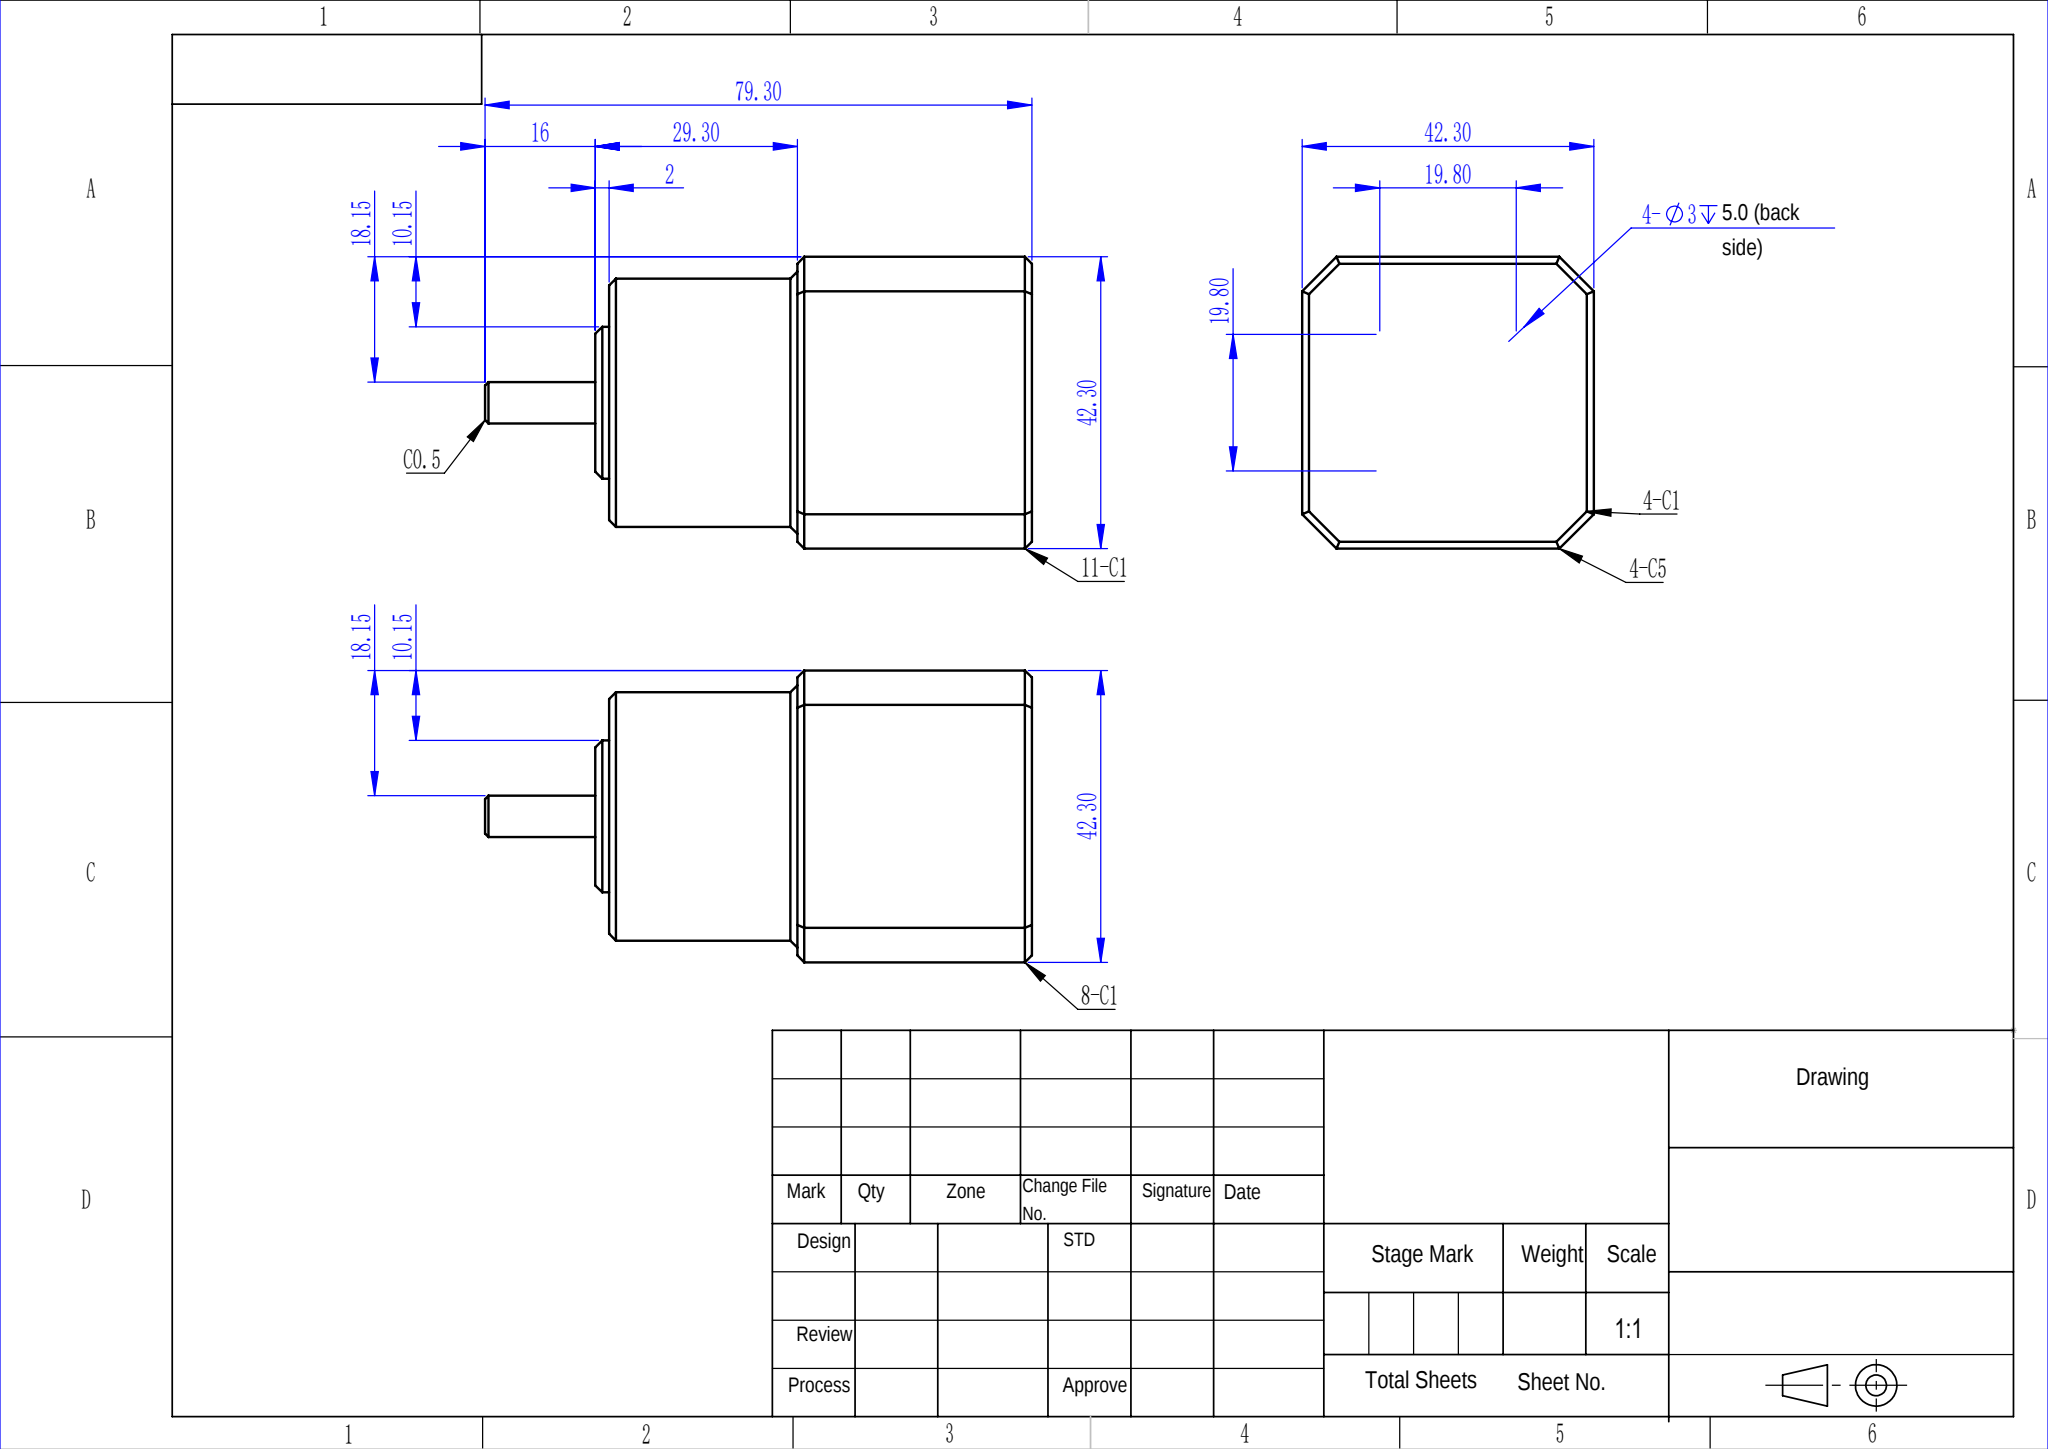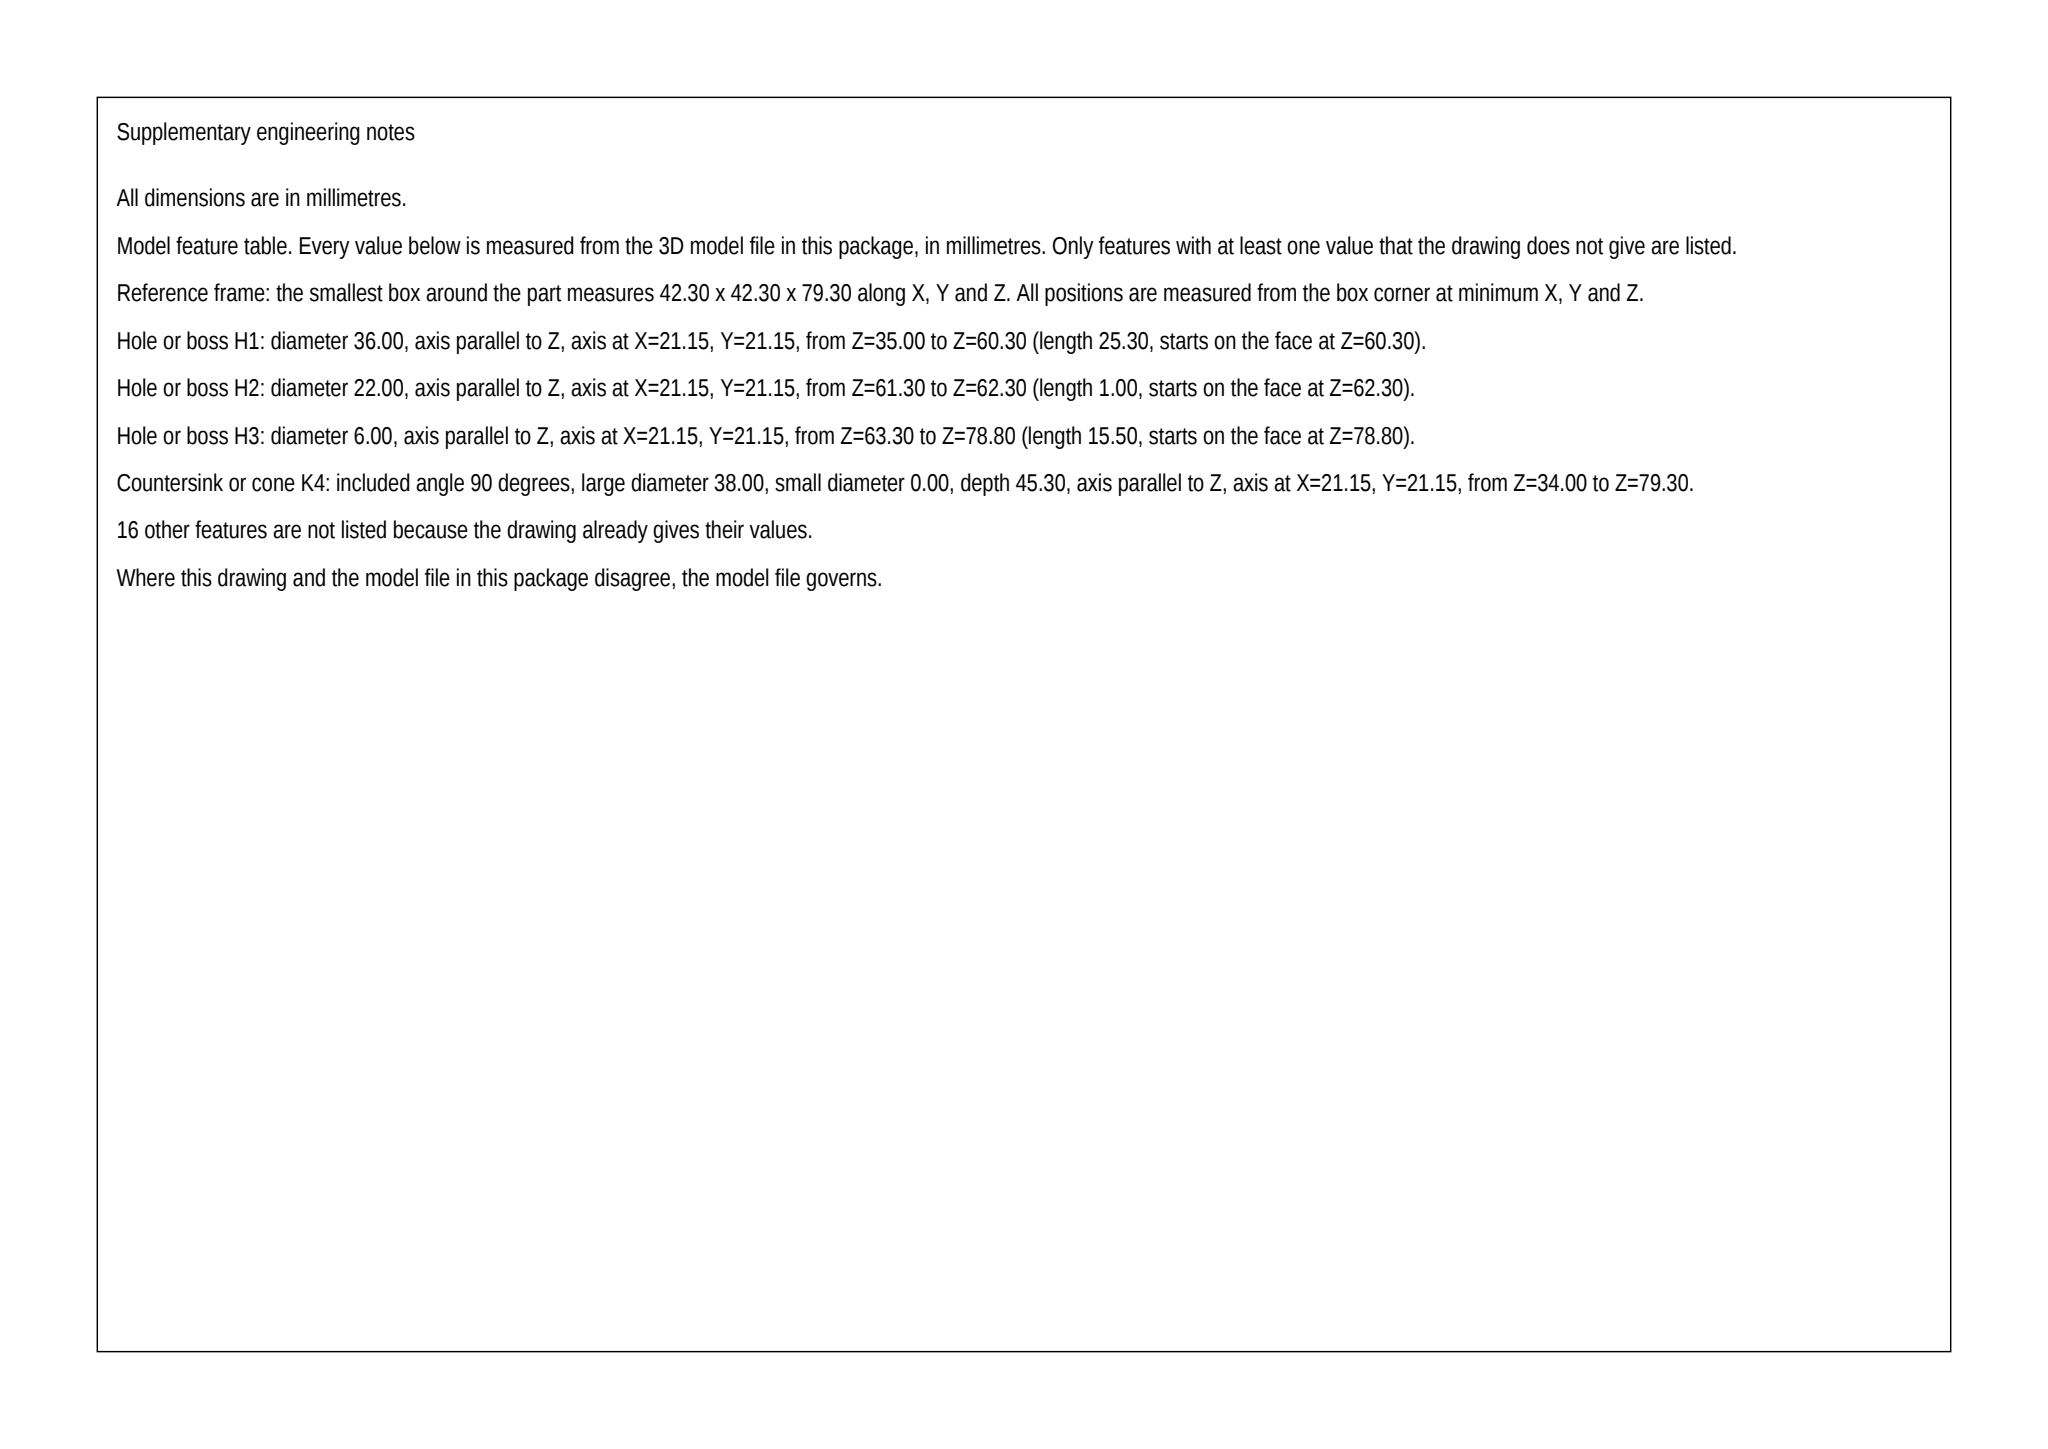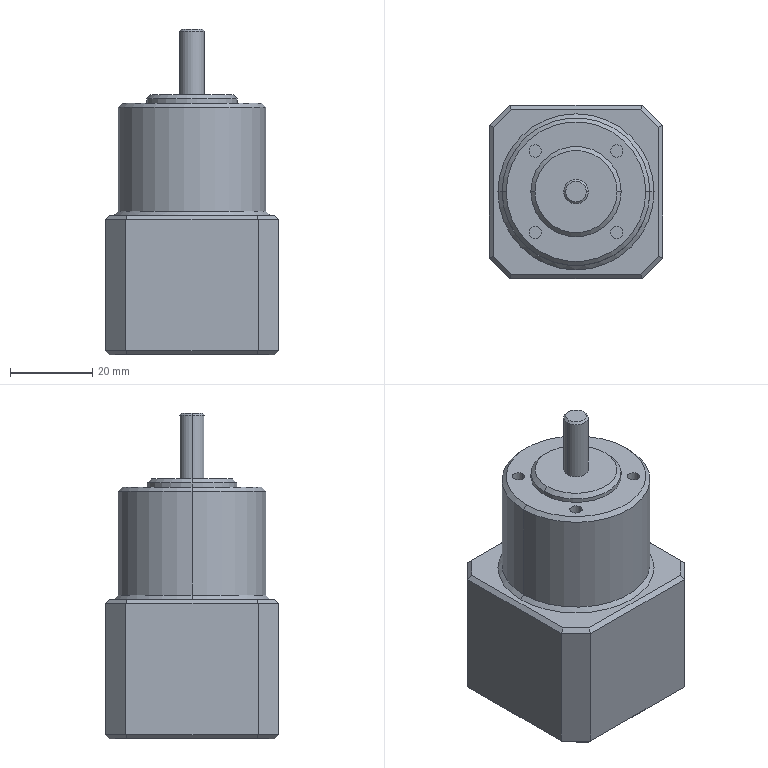Part | SolidWorks | mm | 1 solid | 55 faces | box 42.3 x 42.3 x 79.3 mm | volume 87806 mm3 | plane 33 | cylinder 14 | cone 8 | commonest cylinder face diameters 3 x8 6 x2 22 x2 36 x2
build123d program:
from build123d import *

# Parameters (mm, degrees)
SKETCH1_W           = 42.3
SKETCH1_H           = 42.3
BOSS_EXTRUDE1_DEPTH = 34
CHAMFER1_SIZE       = 5
SKETCH2_R           = 18
BOSS_EXTRUDE2_DEPTH = 27.3
SKETCH3_R           = 11
BOSS_EXTRUDE3_DEPTH = 2
SKETCH4_R           = 3
BOSS_EXTRUDE4_DEPTH = 16
CHAMFER2_SIZE       = 1
CHAMFER3_SIZE       = 0.5
SKETCH5_R           = 1.5
CUT_EXTRUDE1_DEPTH  = 5


with BuildPart() as part:
    # Sketch1 → Boss-Extrude1 (new body)
    with BuildSketch(Plane.XY):
        Rectangle(SKETCH1_W, SKETCH1_H)
    extrude(amount=BOSS_EXTRUDE1_DEPTH)

    # Chamfer1
    chamfer1_edges = [part.edges().sort_by_distance(p)[0] for p in [
        (21.15, -21.15, 17),
        (-21.15, -21.15, 17),
        (-21.15, 21.15, 17),
        (21.15, 21.15, 17),
    ]]
    chamfer(chamfer1_edges, length=CHAMFER1_SIZE)

    # Sketch2 → Boss-Extrude2 (add)
    with BuildSketch(Plane.XY.offset(34)):
        Circle(SKETCH2_R)
    extrude(amount=BOSS_EXTRUDE2_DEPTH)

    # Sketch3 → Boss-Extrude3 (add)
    with BuildSketch(Plane.XY.offset(61.3)):
        Circle(SKETCH3_R)
    extrude(amount=BOSS_EXTRUDE3_DEPTH)

    # Sketch4 → Boss-Extrude4 (add)
    with BuildSketch(Plane.XY.offset(63.3)):
        Circle(SKETCH4_R)
    extrude(amount=BOSS_EXTRUDE4_DEPTH)

    # Chamfer2
    chamfer2_edges = [part.edges().sort_by_distance(p)[0] for p in [
        (0, -21.15, 0),
        (0, -21.15, 34),
        (21.15, 0, 0),
        (-21.15, 0, 0),
        (0, 21.15, 0),
        (18.65, 18.65, 0),
        (18.65, -18.65, 0),
        (-18.65, 18.65, 0),
        (-18.65, -18.65, 0),
        (-21.15, 0, 34),
        (21.15, 0, 34),
        (0, 21.15, 34),
        (18.65, 18.65, 34),
        (18.65, -18.65, 34),
        (-18.65, 18.65, 34),
        (-18.65, -18.65, 34),
        (-18, 0, 34),
        (-18, 0, 61.3),
        (-11, 0, 63.3),
    ]]
    chamfer(chamfer2_edges, length=CHAMFER2_SIZE)

    # Chamfer3
    chamfer3_edges = [part.edges().sort_by_distance(p)[0] for p in [
        (-3, 0, 79.3),
    ]]
    chamfer(chamfer3_edges, length=CHAMFER3_SIZE)

    # Sketch5 → Cut-Extrude1 (cut)
    with BuildSketch(Plane.XY.offset(61.3)):
        with Locations((9.899, 9.899)):
            Circle(SKETCH5_R)
        with Locations((9.899, -9.899)):
            Circle(SKETCH5_R)
        with Locations((-9.899, -9.899)):
            Circle(SKETCH5_R)
        with Locations((-9.899, 9.899)):
            Circle(SKETCH5_R)
    extrude(amount=-CUT_EXTRUDE1_DEPTH, mode=Mode.SUBTRACT)


solid = part.part